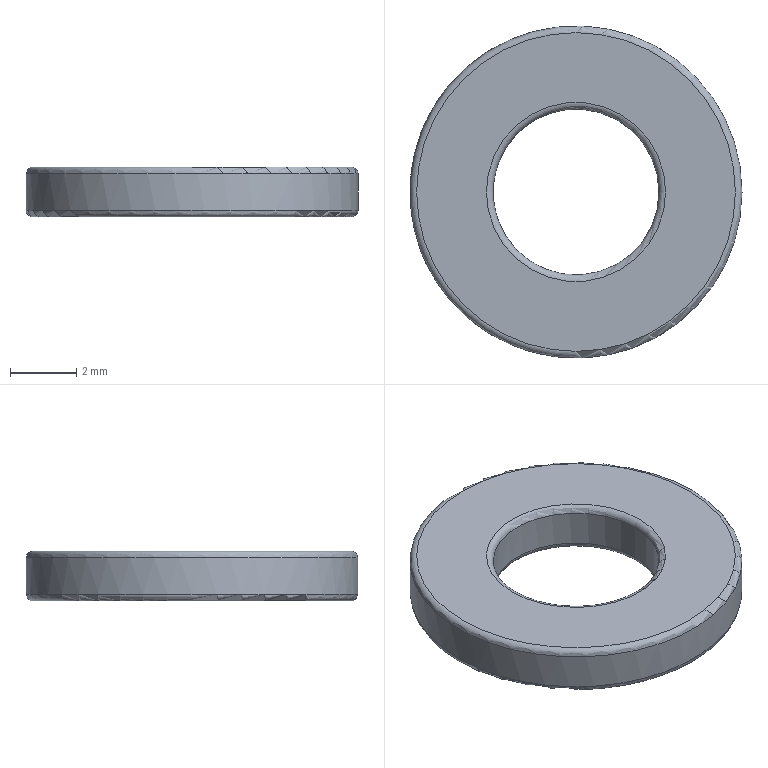Component | NX | MOUNTINGWASHER | 1 solid | 8 faces | box 10 x 10 x 1.5 mm | volume 88 mm3 | torus 4 | plane 2 | cylinder 2 | commonest cylinder face diameters 10 x1 5 x1
STEP:
#1=CARTESIAN_POINT('',(0.,0.,0.));
#2=DIRECTION('',(0.,0.,1.));
#3=DIRECTION('',(1.,0.,0.));
#4=AXIS2_PLACEMENT_3D('',#1,#2,#3);
#5=CARTESIAN_POINT('',(-465.,-20.638,-6.5));
#6=VERTEX_POINT('',#5);
#7=CARTESIAN_POINT('',(-462.3,-20.638,-6.5));
#8=DIRECTION('',(0.,0.,1.));
#9=DIRECTION('',(-1.,0.,0.));
#10=AXIS2_PLACEMENT_3D('',#7,#8,#9);
#11=CIRCLE('',#10,2.7);
#12=CARTESIAN_POINT('',(-462.3,-20.638,-6.5));
#13=DIRECTION('',(0.,0.,-1.));
#14=DIRECTION('',(-1.,0.,0.));
#15=AXIS2_PLACEMENT_3D('',#12,#13,#14);
#16=PLANE('',#15);
#17=CARTESIAN_POINT('',(2.7,0.));
#18=CARTESIAN_POINT('',(2.7,-4.677));
#19=CARTESIAN_POINT('',(-1.35,-2.338));
#20=CARTESIAN_POINT('',(-5.4,-0.));
#21=CARTESIAN_POINT('',(-1.35,2.338));
#22=CARTESIAN_POINT('',(2.7,4.677));
#23=CARTESIAN_POINT('',(2.7,0.));
#24=(BOUNDED_CURVE()B_SPLINE_CURVE(2,(#17,#18,#19,#20,#21,#22,#23),.UNSPECIFIED.,.T.,.F.)B_SPLINE_CURVE_WITH_KNOTS((1,2,2,2,2,1),(-2.094,0.,2.094,4.189,6.283,8.378),.UNSPECIFIED.)CURVE()GEOMETRIC_REPRESENTATION_ITEM()RATIONAL_B_SPLINE_CURVE((1.,0.5,1.,0.5,1.,0.5,1.))REPRESENTATION_ITEM(''));
#25=(GEOMETRIC_REPRESENTATION_CONTEXT(2)PARAMETRIC_REPRESENTATION_CONTEXT()REPRESENTATION_CONTEXT('',''));
#26=DEFINITIONAL_REPRESENTATION('',(#24),#25);
#27=PCURVE('',#16,#26);
#28=CARTESIAN_POINT('',(-462.3,-20.638,-6.3));
#29=DIRECTION('',(0.,0.,-1.));
#30=DIRECTION('',(-1.,0.,0.));
#31=AXIS2_PLACEMENT_3D('',#28,#29,#30);
#32=TOROIDAL_SURFACE('',#31,2.7,0.2);
#33=CARTESIAN_POINT('',(6.283,7.854));
#34=DIRECTION('',(-1.,0.));
#35=VECTOR('',#34,1.);
#36=LINE('',#33,#35);
#37=(GEOMETRIC_REPRESENTATION_CONTEXT(2)PARAMETRIC_REPRESENTATION_CONTEXT()REPRESENTATION_CONTEXT('',''));
#38=DEFINITIONAL_REPRESENTATION('',(#36),#37);
#39=PCURVE('',#32,#38);
#40=SURFACE_CURVE('',#11,(#27,#39),.PCURVE_S1.);
#41=EDGE_CURVE('',#6,#6,#40,.T.);
#42=ORIENTED_EDGE('',*,*,#41,.T.);
#43=EDGE_LOOP('',(#42));
#44=FACE_BOUND('',#43,.T.);
#45=CARTESIAN_POINT('',(-467.1,-20.638,-6.5));
#46=VERTEX_POINT('',#45);
#47=CARTESIAN_POINT('',(-462.3,-20.638,-6.5));
#48=DIRECTION('',(0.,0.,-1.));
#49=DIRECTION('',(-1.,0.,0.));
#50=AXIS2_PLACEMENT_3D('',#47,#48,#49);
#51=CIRCLE('',#50,4.8);
#52=CARTESIAN_POINT('',(0.,0.));
#53=DIRECTION('',(1.,0.));
#54=AXIS2_PLACEMENT_2D('',#52,#53);
#55=CIRCLE('',#54,4.8);
#56=(GEOMETRIC_REPRESENTATION_CONTEXT(2)PARAMETRIC_REPRESENTATION_CONTEXT()REPRESENTATION_CONTEXT('',''));
#57=DEFINITIONAL_REPRESENTATION('',(#55),#56);
#58=PCURVE('',#16,#57);
#59=CARTESIAN_POINT('',(-462.3,-20.638,-6.3));
#60=DIRECTION('',(0.,0.,-1.));
#61=DIRECTION('',(-1.,0.,0.));
#62=AXIS2_PLACEMENT_3D('',#59,#60,#61);
#63=TOROIDAL_SURFACE('',#62,4.8,0.2);
#64=CARTESIAN_POINT('',(0.,7.854));
#65=DIRECTION('',(1.,0.));
#66=VECTOR('',#65,1.);
#67=LINE('',#64,#66);
#68=(GEOMETRIC_REPRESENTATION_CONTEXT(2)PARAMETRIC_REPRESENTATION_CONTEXT()REPRESENTATION_CONTEXT('',''));
#69=DEFINITIONAL_REPRESENTATION('',(#67),#68);
#70=PCURVE('',#63,#69);
#71=SURFACE_CURVE('',#51,(#58,#70),.PCURVE_S1.);
#72=EDGE_CURVE('',#46,#46,#71,.T.);
#73=ORIENTED_EDGE('',*,*,#72,.T.);
#74=EDGE_LOOP('',(#73));
#75=FACE_BOUND('',#74,.T.);
#76=ADVANCED_FACE('',(#44,#75),#16,.T.);
#77=CARTESIAN_POINT('',(-459.6,-20.638,-5.));
#78=VERTEX_POINT('',#77);
#79=CARTESIAN_POINT('',(-462.3,-20.638,-5.));
#80=DIRECTION('',(0.,0.,-1.));
#81=DIRECTION('',(1.,0.,0.));
#82=AXIS2_PLACEMENT_3D('',#79,#80,#81);
#83=CIRCLE('',#82,2.7);
#84=CARTESIAN_POINT('',(-462.3,-20.638,-5.));
#85=DIRECTION('',(0.,0.,1.));
#86=DIRECTION('',(1.,0.,0.));
#87=AXIS2_PLACEMENT_3D('',#84,#85,#86);
#88=PLANE('',#87);
#89=CARTESIAN_POINT('',(2.7,0.));
#90=CARTESIAN_POINT('',(2.7,-4.677));
#91=CARTESIAN_POINT('',(-1.35,-2.338));
#92=CARTESIAN_POINT('',(-5.4,-0.));
#93=CARTESIAN_POINT('',(-1.35,2.338));
#94=CARTESIAN_POINT('',(2.7,4.677));
#95=CARTESIAN_POINT('',(2.7,0.));
#96=(BOUNDED_CURVE()B_SPLINE_CURVE(2,(#89,#90,#91,#92,#93,#94,#95),.UNSPECIFIED.,.T.,.F.)B_SPLINE_CURVE_WITH_KNOTS((1,2,2,2,2,1),(-2.094,0.,2.094,4.189,6.283,8.378),.UNSPECIFIED.)CURVE()GEOMETRIC_REPRESENTATION_ITEM()RATIONAL_B_SPLINE_CURVE((1.,0.5,1.,0.5,1.,0.5,1.))REPRESENTATION_ITEM(''));
#97=(GEOMETRIC_REPRESENTATION_CONTEXT(2)PARAMETRIC_REPRESENTATION_CONTEXT()REPRESENTATION_CONTEXT('',''));
#98=DEFINITIONAL_REPRESENTATION('',(#96),#97);
#99=PCURVE('',#88,#98);
#100=CARTESIAN_POINT('',(-462.3,-20.638,-5.2));
#101=DIRECTION('',(0.,0.,1.));
#102=DIRECTION('',(1.,0.,0.));
#103=AXIS2_PLACEMENT_3D('',#100,#101,#102);
#104=TOROIDAL_SURFACE('',#103,2.7,0.2);
#105=CARTESIAN_POINT('',(6.283,7.854));
#106=DIRECTION('',(-1.,0.));
#107=VECTOR('',#106,1.);
#108=LINE('',#105,#107);
#109=(GEOMETRIC_REPRESENTATION_CONTEXT(2)PARAMETRIC_REPRESENTATION_CONTEXT()REPRESENTATION_CONTEXT('',''));
#110=DEFINITIONAL_REPRESENTATION('',(#108),#109);
#111=PCURVE('',#104,#110);
#112=SURFACE_CURVE('',#83,(#99,#111),.PCURVE_S1.);
#113=EDGE_CURVE('',#78,#78,#112,.T.);
#114=ORIENTED_EDGE('',*,*,#113,.T.);
#115=EDGE_LOOP('',(#114));
#116=FACE_BOUND('',#115,.T.);
#117=CARTESIAN_POINT('',(-457.5,-20.638,-5.));
#118=VERTEX_POINT('',#117);
#119=CARTESIAN_POINT('',(-462.3,-20.638,-5.));
#120=DIRECTION('',(0.,0.,1.));
#121=DIRECTION('',(1.,0.,0.));
#122=AXIS2_PLACEMENT_3D('',#119,#120,#121);
#123=CIRCLE('',#122,4.8);
#124=CARTESIAN_POINT('',(0.,0.));
#125=DIRECTION('',(1.,0.));
#126=AXIS2_PLACEMENT_2D('',#124,#125);
#127=CIRCLE('',#126,4.8);
#128=(GEOMETRIC_REPRESENTATION_CONTEXT(2)PARAMETRIC_REPRESENTATION_CONTEXT()REPRESENTATION_CONTEXT('',''));
#129=DEFINITIONAL_REPRESENTATION('',(#127),#128);
#130=PCURVE('',#88,#129);
#131=CARTESIAN_POINT('',(-462.3,-20.638,-5.2));
#132=DIRECTION('',(0.,0.,1.));
#133=DIRECTION('',(1.,0.,0.));
#134=AXIS2_PLACEMENT_3D('',#131,#132,#133);
#135=TOROIDAL_SURFACE('',#134,4.8,0.2);
#136=CARTESIAN_POINT('',(0.,7.854));
#137=DIRECTION('',(1.,0.));
#138=VECTOR('',#137,1.);
#139=LINE('',#136,#138);
#140=(GEOMETRIC_REPRESENTATION_CONTEXT(2)PARAMETRIC_REPRESENTATION_CONTEXT()REPRESENTATION_CONTEXT('',''));
#141=DEFINITIONAL_REPRESENTATION('',(#139),#140);
#142=PCURVE('',#135,#141);
#143=SURFACE_CURVE('',#123,(#130,#142),.PCURVE_S1.);
#144=EDGE_CURVE('',#118,#118,#143,.T.);
#145=ORIENTED_EDGE('',*,*,#144,.T.);
#146=EDGE_LOOP('',(#145));
#147=FACE_BOUND('',#146,.T.);
#148=ADVANCED_FACE('',(#116,#147),#88,.T.);
#149=CARTESIAN_POINT('',(-457.3,-20.638,-5.2));
#150=VERTEX_POINT('',#149);
#151=CARTESIAN_POINT('',(-462.3,-20.638,-5.2));
#152=DIRECTION('',(0.,0.,-1.));
#153=DIRECTION('',(1.,0.,0.));
#154=AXIS2_PLACEMENT_3D('',#151,#152,#153);
#155=CIRCLE('',#154,5.);
#156=CARTESIAN_POINT('',(-462.3,-20.638,-5.));
#157=DIRECTION('',(0.,0.,-1.));
#158=DIRECTION('',(1.,0.,0.));
#159=AXIS2_PLACEMENT_3D('',#156,#157,#158);
#160=CYLINDRICAL_SURFACE('',#159,5.);
#161=CARTESIAN_POINT('',(0.,0.2));
#162=DIRECTION('',(1.,0.));
#163=VECTOR('',#162,1.);
#164=LINE('',#161,#163);
#165=(GEOMETRIC_REPRESENTATION_CONTEXT(2)PARAMETRIC_REPRESENTATION_CONTEXT()REPRESENTATION_CONTEXT('',''));
#166=DEFINITIONAL_REPRESENTATION('',(#164),#165);
#167=PCURVE('',#160,#166);
#168=CARTESIAN_POINT('',(6.283,6.283));
#169=DIRECTION('',(-1.,0.));
#170=VECTOR('',#169,1.);
#171=LINE('',#168,#170);
#172=(GEOMETRIC_REPRESENTATION_CONTEXT(2)PARAMETRIC_REPRESENTATION_CONTEXT()REPRESENTATION_CONTEXT('',''));
#173=DEFINITIONAL_REPRESENTATION('',(#171),#172);
#174=PCURVE('',#135,#173);
#175=SURFACE_CURVE('',#155,(#167,#174),.PCURVE_S1.);
#176=EDGE_CURVE('',#150,#150,#175,.T.);
#177=ORIENTED_EDGE('',*,*,#176,.T.);
#178=CARTESIAN_POINT('',(-457.3,-20.638,-6.3));
#179=VERTEX_POINT('',#178);
#180=CARTESIAN_POINT('',(-457.3,-20.638,-5.2));
#181=CARTESIAN_POINT('',(-457.3,-20.638,-6.3));
#182=B_SPLINE_CURVE_WITH_KNOTS('',1,(#180,#181),.UNSPECIFIED.,.F.,.F.,(2,2),(0.2,1.3),.PIECEWISE_BEZIER_KNOTS.);
#183=CARTESIAN_POINT('',(6.283,0.));
#184=DIRECTION('',(0.,1.));
#185=VECTOR('',#184,1.);
#186=LINE('',#183,#185);
#187=(GEOMETRIC_REPRESENTATION_CONTEXT(2)PARAMETRIC_REPRESENTATION_CONTEXT()REPRESENTATION_CONTEXT('',''));
#188=DEFINITIONAL_REPRESENTATION('',(#186),#187);
#189=PCURVE('',#160,#188);
#190=CARTESIAN_POINT('',(0.,0.));
#191=DIRECTION('',(0.,1.));
#192=VECTOR('',#191,1.);
#193=LINE('',#190,#192);
#194=(GEOMETRIC_REPRESENTATION_CONTEXT(2)PARAMETRIC_REPRESENTATION_CONTEXT()REPRESENTATION_CONTEXT('',''));
#195=DEFINITIONAL_REPRESENTATION('',(#193),#194);
#196=PCURVE('',#160,#195);
#197=SEAM_CURVE('',#182,(#189,#196),.PCURVE_S1.);
#198=EDGE_CURVE('',#150,#179,#197,.T.);
#199=ORIENTED_EDGE('',*,*,#198,.T.);
#200=CARTESIAN_POINT('',(-467.3,-20.638,-6.3));
#201=VERTEX_POINT('',#200);
#202=CARTESIAN_POINT('',(-462.3,-20.638,-6.3));
#203=DIRECTION('',(0.,0.,1.));
#204=DIRECTION('',(-1.,0.,0.));
#205=AXIS2_PLACEMENT_3D('',#202,#203,#204);
#206=CIRCLE('',#205,5.);
#207=CARTESIAN_POINT('',(9.425,1.3));
#208=DIRECTION('',(-1.,0.));
#209=VECTOR('',#208,1.);
#210=LINE('',#207,#209);
#211=(GEOMETRIC_REPRESENTATION_CONTEXT(2)PARAMETRIC_REPRESENTATION_CONTEXT()REPRESENTATION_CONTEXT('',''));
#212=DEFINITIONAL_REPRESENTATION('',(#210),#211);
#213=PCURVE('',#160,#212);
#214=CARTESIAN_POINT('',(6.283,6.283));
#215=DIRECTION('',(-1.,0.));
#216=VECTOR('',#215,1.);
#217=LINE('',#214,#216);
#218=(GEOMETRIC_REPRESENTATION_CONTEXT(2)PARAMETRIC_REPRESENTATION_CONTEXT()REPRESENTATION_CONTEXT('',''));
#219=DEFINITIONAL_REPRESENTATION('',(#217),#218);
#220=PCURVE('',#63,#219);
#221=SURFACE_CURVE('',#206,(#213,#220),.PCURVE_S1.);
#222=EDGE_CURVE('',#179,#201,#221,.T.);
#223=ORIENTED_EDGE('',*,*,#222,.T.);
#224=CARTESIAN_POINT('',(-462.3,-20.638,-6.3));
#225=DIRECTION('',(0.,0.,1.));
#226=DIRECTION('',(-1.,0.,0.));
#227=AXIS2_PLACEMENT_3D('',#224,#225,#226);
#228=CIRCLE('',#227,5.);
#229=CARTESIAN_POINT('',(3.142,1.3));
#230=DIRECTION('',(-1.,0.));
#231=VECTOR('',#230,1.);
#232=LINE('',#229,#231);
#233=(GEOMETRIC_REPRESENTATION_CONTEXT(2)PARAMETRIC_REPRESENTATION_CONTEXT()REPRESENTATION_CONTEXT('',''));
#234=DEFINITIONAL_REPRESENTATION('',(#232),#233);
#235=PCURVE('',#160,#234);
#236=CARTESIAN_POINT('',(6.283,6.283));
#237=DIRECTION('',(-1.,0.));
#238=VECTOR('',#237,1.);
#239=LINE('',#236,#238);
#240=(GEOMETRIC_REPRESENTATION_CONTEXT(2)PARAMETRIC_REPRESENTATION_CONTEXT()REPRESENTATION_CONTEXT('',''));
#241=DEFINITIONAL_REPRESENTATION('',(#239),#240);
#242=PCURVE('',#63,#241);
#243=SURFACE_CURVE('',#228,(#235,#242),.PCURVE_S1.);
#244=EDGE_CURVE('',#201,#179,#243,.T.);
#245=ORIENTED_EDGE('',*,*,#244,.T.);
#246=ORIENTED_EDGE('',*,*,#198,.F.);
#247=EDGE_LOOP('',(#177,#199,#223,#245,#246));
#248=FACE_BOUND('',#247,.T.);
#249=ADVANCED_FACE('',(#248),#160,.T.);
#250=CARTESIAN_POINT('',(-459.8,-20.638,-6.3));
#251=VERTEX_POINT('',#250);
#252=CARTESIAN_POINT('',(-464.8,-20.638,-6.3));
#253=VERTEX_POINT('',#252);
#254=CARTESIAN_POINT('',(-462.3,-20.638,-6.3));
#255=DIRECTION('',(0.,0.,-1.));
#256=DIRECTION('',(-1.,0.,0.));
#257=AXIS2_PLACEMENT_3D('',#254,#255,#256);
#258=CIRCLE('',#257,2.5);
#259=CARTESIAN_POINT('',(-462.3,-20.638,-6.5));
#260=DIRECTION('',(0.,0.,1.));
#261=DIRECTION('',(1.,0.,0.));
#262=AXIS2_PLACEMENT_3D('',#259,#260,#261);
#263=CYLINDRICAL_SURFACE('',#262,2.5);
#264=CARTESIAN_POINT('',(9.425,0.2));
#265=DIRECTION('',(-1.,0.));
#266=VECTOR('',#265,1.);
#267=LINE('',#264,#266);
#268=(GEOMETRIC_REPRESENTATION_CONTEXT(2)PARAMETRIC_REPRESENTATION_CONTEXT()REPRESENTATION_CONTEXT('',''));
#269=DEFINITIONAL_REPRESENTATION('',(#267),#268);
#270=PCURVE('',#263,#269);
#271=CARTESIAN_POINT('',(0.,9.425));
#272=DIRECTION('',(1.,0.));
#273=VECTOR('',#272,1.);
#274=LINE('',#271,#273);
#275=(GEOMETRIC_REPRESENTATION_CONTEXT(2)PARAMETRIC_REPRESENTATION_CONTEXT()REPRESENTATION_CONTEXT('',''));
#276=DEFINITIONAL_REPRESENTATION('',(#274),#275);
#277=PCURVE('',#32,#276);
#278=SURFACE_CURVE('',#258,(#270,#277),.PCURVE_S1.);
#279=EDGE_CURVE('',#251,#253,#278,.T.);
#280=ORIENTED_EDGE('',*,*,#279,.F.);
#281=CARTESIAN_POINT('',(-459.8,-20.638,-5.2));
#282=VERTEX_POINT('',#281);
#283=CARTESIAN_POINT('',(-459.8,-20.638,-6.3));
#284=CARTESIAN_POINT('',(-459.8,-20.638,-5.2));
#285=B_SPLINE_CURVE_WITH_KNOTS('',1,(#283,#284),.UNSPECIFIED.,.F.,.F.,(2,2),(0.2,1.3),.PIECEWISE_BEZIER_KNOTS.);
#286=CARTESIAN_POINT('',(6.283,0.));
#287=DIRECTION('',(0.,1.));
#288=VECTOR('',#287,1.);
#289=LINE('',#286,#288);
#290=(GEOMETRIC_REPRESENTATION_CONTEXT(2)PARAMETRIC_REPRESENTATION_CONTEXT()REPRESENTATION_CONTEXT('',''));
#291=DEFINITIONAL_REPRESENTATION('',(#289),#290);
#292=PCURVE('',#263,#291);
#293=CARTESIAN_POINT('',(0.,0.));
#294=DIRECTION('',(0.,1.));
#295=VECTOR('',#294,1.);
#296=LINE('',#293,#295);
#297=(GEOMETRIC_REPRESENTATION_CONTEXT(2)PARAMETRIC_REPRESENTATION_CONTEXT()REPRESENTATION_CONTEXT('',''));
#298=DEFINITIONAL_REPRESENTATION('',(#296),#297);
#299=PCURVE('',#263,#298);
#300=SEAM_CURVE('',#285,(#292,#299),.PCURVE_S1.);
#301=EDGE_CURVE('',#251,#282,#300,.T.);
#302=ORIENTED_EDGE('',*,*,#301,.T.);
#303=CARTESIAN_POINT('',(-462.3,-20.638,-5.2));
#304=DIRECTION('',(0.,0.,1.));
#305=DIRECTION('',(1.,0.,0.));
#306=AXIS2_PLACEMENT_3D('',#303,#304,#305);
#307=CIRCLE('',#306,2.5);
#308=CARTESIAN_POINT('',(0.,1.3));
#309=DIRECTION('',(1.,0.));
#310=VECTOR('',#309,1.);
#311=LINE('',#308,#310);
#312=(GEOMETRIC_REPRESENTATION_CONTEXT(2)PARAMETRIC_REPRESENTATION_CONTEXT()REPRESENTATION_CONTEXT('',''));
#313=DEFINITIONAL_REPRESENTATION('',(#311),#312);
#314=PCURVE('',#263,#313);
#315=CARTESIAN_POINT('',(0.,9.425));
#316=DIRECTION('',(1.,0.));
#317=VECTOR('',#316,1.);
#318=LINE('',#315,#317);
#319=(GEOMETRIC_REPRESENTATION_CONTEXT(2)PARAMETRIC_REPRESENTATION_CONTEXT()REPRESENTATION_CONTEXT('',''));
#320=DEFINITIONAL_REPRESENTATION('',(#318),#319);
#321=PCURVE('',#104,#320);
#322=SURFACE_CURVE('',#307,(#314,#321),.PCURVE_S1.);
#323=EDGE_CURVE('',#282,#282,#322,.T.);
#324=ORIENTED_EDGE('',*,*,#323,.F.);
#325=ORIENTED_EDGE('',*,*,#301,.F.);
#326=CARTESIAN_POINT('',(-462.3,-20.638,-6.3));
#327=DIRECTION('',(0.,0.,-1.));
#328=DIRECTION('',(-1.,0.,0.));
#329=AXIS2_PLACEMENT_3D('',#326,#327,#328);
#330=CIRCLE('',#329,2.5);
#331=CARTESIAN_POINT('',(3.142,0.2));
#332=DIRECTION('',(-1.,0.));
#333=VECTOR('',#332,1.);
#334=LINE('',#331,#333);
#335=(GEOMETRIC_REPRESENTATION_CONTEXT(2)PARAMETRIC_REPRESENTATION_CONTEXT()REPRESENTATION_CONTEXT('',''));
#336=DEFINITIONAL_REPRESENTATION('',(#334),#335);
#337=PCURVE('',#263,#336);
#338=CARTESIAN_POINT('',(0.,9.425));
#339=DIRECTION('',(1.,-0.));
#340=VECTOR('',#339,1.);
#341=LINE('',#338,#340);
#342=(GEOMETRIC_REPRESENTATION_CONTEXT(2)PARAMETRIC_REPRESENTATION_CONTEXT()REPRESENTATION_CONTEXT('',''));
#343=DEFINITIONAL_REPRESENTATION('',(#341),#342);
#344=PCURVE('',#32,#343);
#345=SURFACE_CURVE('',#330,(#337,#344),.PCURVE_S1.);
#346=EDGE_CURVE('',#253,#251,#345,.T.);
#347=ORIENTED_EDGE('',*,*,#346,.F.);
#348=EDGE_LOOP('',(#280,#302,#324,#325,#347));
#349=FACE_BOUND('',#348,.F.);
#350=ADVANCED_FACE('',(#349),#263,.F.);
#351=ORIENTED_EDGE('',*,*,#346,.F.);
#352=CARTESIAN_POINT('',(-465.,-20.638,-6.5));
#353=CARTESIAN_POINT('',(-464.947,-20.638,-6.5));
#354=CARTESIAN_POINT('',(-464.894,-20.638,-6.483));
#355=CARTESIAN_POINT('',(-464.85,-20.638,-6.45));
#356=CARTESIAN_POINT('',(-464.817,-20.638,-6.406));
#357=CARTESIAN_POINT('',(-464.8,-20.638,-6.353));
#358=CARTESIAN_POINT('',(-464.8,-20.638,-6.3));
#359=(BOUNDED_CURVE()B_SPLINE_CURVE(6,(#352,#353,#354,#355,#356,#357,#358),.UNSPECIFIED.,.F.,.F.)B_SPLINE_CURVE_WITH_KNOTS((7,7),(1.571,3.142),.PIECEWISE_BEZIER_KNOTS.)CURVE()GEOMETRIC_REPRESENTATION_ITEM()RATIONAL_B_SPLINE_CURVE((1.031,1.01,0.9979,0.994,0.9979,1.01,1.031))REPRESENTATION_ITEM(''));
#360=CARTESIAN_POINT('',(0.,6.283));
#361=DIRECTION('',(0.,1.));
#362=VECTOR('',#361,1.);
#363=LINE('',#360,#362);
#364=(GEOMETRIC_REPRESENTATION_CONTEXT(2)PARAMETRIC_REPRESENTATION_CONTEXT()REPRESENTATION_CONTEXT('',''));
#365=DEFINITIONAL_REPRESENTATION('',(#363),#364);
#366=PCURVE('',#32,#365);
#367=CARTESIAN_POINT('',(6.283,6.283));
#368=DIRECTION('',(0.,1.));
#369=VECTOR('',#368,1.);
#370=LINE('',#367,#369);
#371=(GEOMETRIC_REPRESENTATION_CONTEXT(2)PARAMETRIC_REPRESENTATION_CONTEXT()REPRESENTATION_CONTEXT('',''));
#372=DEFINITIONAL_REPRESENTATION('',(#370),#371);
#373=PCURVE('',#32,#372);
#374=SEAM_CURVE('',#359,(#366,#373),.PCURVE_S1.);
#375=EDGE_CURVE('',#6,#253,#374,.T.);
#376=ORIENTED_EDGE('',*,*,#375,.F.);
#377=ORIENTED_EDGE('',*,*,#41,.F.);
#378=ORIENTED_EDGE('',*,*,#375,.T.);
#379=ORIENTED_EDGE('',*,*,#279,.F.);
#380=EDGE_LOOP('',(#351,#376,#377,#378,#379));
#381=FACE_BOUND('',#380,.T.);
#382=ADVANCED_FACE('',(#381),#32,.T.);
#383=ORIENTED_EDGE('',*,*,#323,.F.);
#384=CARTESIAN_POINT('',(-459.6,-20.638,-5.));
#385=CARTESIAN_POINT('',(-459.653,-20.638,-5.));
#386=CARTESIAN_POINT('',(-459.706,-20.638,-5.017));
#387=CARTESIAN_POINT('',(-459.75,-20.638,-5.05));
#388=CARTESIAN_POINT('',(-459.783,-20.638,-5.094));
#389=CARTESIAN_POINT('',(-459.8,-20.638,-5.147));
#390=CARTESIAN_POINT('',(-459.8,-20.638,-5.2));
#391=(BOUNDED_CURVE()B_SPLINE_CURVE(6,(#384,#385,#386,#387,#388,#389,#390),.UNSPECIFIED.,.F.,.F.)B_SPLINE_CURVE_WITH_KNOTS((7,7),(1.571,3.142),.PIECEWISE_BEZIER_KNOTS.)CURVE()GEOMETRIC_REPRESENTATION_ITEM()RATIONAL_B_SPLINE_CURVE((1.031,1.01,0.9979,0.994,0.9979,1.01,1.031))REPRESENTATION_ITEM(''));
#392=CARTESIAN_POINT('',(0.,6.283));
#393=DIRECTION('',(0.,1.));
#394=VECTOR('',#393,1.);
#395=LINE('',#392,#394);
#396=(GEOMETRIC_REPRESENTATION_CONTEXT(2)PARAMETRIC_REPRESENTATION_CONTEXT()REPRESENTATION_CONTEXT('',''));
#397=DEFINITIONAL_REPRESENTATION('',(#395),#396);
#398=PCURVE('',#104,#397);
#399=CARTESIAN_POINT('',(6.283,6.283));
#400=DIRECTION('',(0.,1.));
#401=VECTOR('',#400,1.);
#402=LINE('',#399,#401);
#403=(GEOMETRIC_REPRESENTATION_CONTEXT(2)PARAMETRIC_REPRESENTATION_CONTEXT()REPRESENTATION_CONTEXT('',''));
#404=DEFINITIONAL_REPRESENTATION('',(#402),#403);
#405=PCURVE('',#104,#404);
#406=SEAM_CURVE('',#391,(#398,#405),.PCURVE_S1.);
#407=EDGE_CURVE('',#78,#282,#406,.T.);
#408=ORIENTED_EDGE('',*,*,#407,.F.);
#409=ORIENTED_EDGE('',*,*,#113,.F.);
#410=ORIENTED_EDGE('',*,*,#407,.T.);
#411=EDGE_LOOP('',(#383,#408,#409,#410));
#412=FACE_BOUND('',#411,.T.);
#413=ADVANCED_FACE('',(#412),#104,.T.);
#414=ORIENTED_EDGE('',*,*,#144,.F.);
#415=CARTESIAN_POINT('',(-457.3,-20.638,-5.2));
#416=CARTESIAN_POINT('',(-457.3,-20.638,-5.147));
#417=CARTESIAN_POINT('',(-457.317,-20.638,-5.094));
#418=CARTESIAN_POINT('',(-457.35,-20.638,-5.05));
#419=CARTESIAN_POINT('',(-457.394,-20.638,-5.017));
#420=CARTESIAN_POINT('',(-457.447,-20.638,-5.));
#421=CARTESIAN_POINT('',(-457.5,-20.638,-5.));
#422=(BOUNDED_CURVE()B_SPLINE_CURVE(6,(#415,#416,#417,#418,#419,#420,#421),.UNSPECIFIED.,.F.,.F.)B_SPLINE_CURVE_WITH_KNOTS((7,7),(0.,1.571),.PIECEWISE_BEZIER_KNOTS.)CURVE()GEOMETRIC_REPRESENTATION_ITEM()RATIONAL_B_SPLINE_CURVE((1.031,1.01,0.9979,0.994,0.9979,1.01,1.031))REPRESENTATION_ITEM(''));
#423=CARTESIAN_POINT('',(0.,6.283));
#424=DIRECTION('',(0.,1.));
#425=VECTOR('',#424,1.);
#426=LINE('',#423,#425);
#427=(GEOMETRIC_REPRESENTATION_CONTEXT(2)PARAMETRIC_REPRESENTATION_CONTEXT()REPRESENTATION_CONTEXT('',''));
#428=DEFINITIONAL_REPRESENTATION('',(#426),#427);
#429=PCURVE('',#135,#428);
#430=CARTESIAN_POINT('',(6.283,6.283));
#431=DIRECTION('',(0.,1.));
#432=VECTOR('',#431,1.);
#433=LINE('',#430,#432);
#434=(GEOMETRIC_REPRESENTATION_CONTEXT(2)PARAMETRIC_REPRESENTATION_CONTEXT()REPRESENTATION_CONTEXT('',''));
#435=DEFINITIONAL_REPRESENTATION('',(#433),#434);
#436=PCURVE('',#135,#435);
#437=SEAM_CURVE('',#422,(#429,#436),.PCURVE_S1.);
#438=EDGE_CURVE('',#150,#118,#437,.T.);
#439=ORIENTED_EDGE('',*,*,#438,.F.);
#440=ORIENTED_EDGE('',*,*,#176,.F.);
#441=ORIENTED_EDGE('',*,*,#438,.T.);
#442=EDGE_LOOP('',(#414,#439,#440,#441));
#443=FACE_BOUND('',#442,.T.);
#444=ADVANCED_FACE('',(#443),#135,.T.);
#445=ORIENTED_EDGE('',*,*,#72,.F.);
#446=CARTESIAN_POINT('',(-467.3,-20.638,-6.3));
#447=CARTESIAN_POINT('',(-467.3,-20.638,-6.353));
#448=CARTESIAN_POINT('',(-467.283,-20.638,-6.406));
#449=CARTESIAN_POINT('',(-467.25,-20.638,-6.45));
#450=CARTESIAN_POINT('',(-467.206,-20.638,-6.483));
#451=CARTESIAN_POINT('',(-467.153,-20.638,-6.5));
#452=CARTESIAN_POINT('',(-467.1,-20.638,-6.5));
#453=(BOUNDED_CURVE()B_SPLINE_CURVE(6,(#446,#447,#448,#449,#450,#451,#452),.UNSPECIFIED.,.F.,.F.)B_SPLINE_CURVE_WITH_KNOTS((7,7),(0.,1.571),.PIECEWISE_BEZIER_KNOTS.)CURVE()GEOMETRIC_REPRESENTATION_ITEM()RATIONAL_B_SPLINE_CURVE((1.031,1.01,0.9979,0.994,0.9979,1.01,1.031))REPRESENTATION_ITEM(''));
#454=CARTESIAN_POINT('',(0.,6.283));
#455=DIRECTION('',(0.,1.));
#456=VECTOR('',#455,1.);
#457=LINE('',#454,#456);
#458=(GEOMETRIC_REPRESENTATION_CONTEXT(2)PARAMETRIC_REPRESENTATION_CONTEXT()REPRESENTATION_CONTEXT('',''));
#459=DEFINITIONAL_REPRESENTATION('',(#457),#458);
#460=PCURVE('',#63,#459);
#461=CARTESIAN_POINT('',(6.283,6.283));
#462=DIRECTION('',(0.,1.));
#463=VECTOR('',#462,1.);
#464=LINE('',#461,#463);
#465=(GEOMETRIC_REPRESENTATION_CONTEXT(2)PARAMETRIC_REPRESENTATION_CONTEXT()REPRESENTATION_CONTEXT('',''));
#466=DEFINITIONAL_REPRESENTATION('',(#464),#465);
#467=PCURVE('',#63,#466);
#468=SEAM_CURVE('',#453,(#460,#467),.PCURVE_S1.);
#469=EDGE_CURVE('',#201,#46,#468,.T.);
#470=ORIENTED_EDGE('',*,*,#469,.F.);
#471=ORIENTED_EDGE('',*,*,#222,.F.);
#472=ORIENTED_EDGE('',*,*,#244,.F.);
#473=ORIENTED_EDGE('',*,*,#469,.T.);
#474=EDGE_LOOP('',(#445,#470,#471,#472,#473));
#475=FACE_BOUND('',#474,.T.);
#476=ADVANCED_FACE('',(#475),#63,.T.);
#477=CLOSED_SHELL('',(#76,#148,#249,#350,#382,#413,#444,#476));
#478=MANIFOLD_SOLID_BREP('',#477);
#479=(LENGTH_UNIT()NAMED_UNIT(*)SI_UNIT(.MILLI.,.METRE.));
#480=UNCERTAINTY_MEASURE_WITH_UNIT(LENGTH_MEASURE(0.00001),#479,'','');
#481=(NAMED_UNIT(*)PLANE_ANGLE_UNIT()SI_UNIT($,.RADIAN.));
#482=(NAMED_UNIT(*)SI_UNIT($,.STERADIAN.)SOLID_ANGLE_UNIT());
#483=(GEOMETRIC_REPRESENTATION_CONTEXT(3)GLOBAL_UNCERTAINTY_ASSIGNED_CONTEXT((#480))GLOBAL_UNIT_ASSIGNED_CONTEXT((#479,#481,#482))REPRESENTATION_CONTEXT('',''));
#484=ADVANCED_BREP_SHAPE_REPRESENTATION('',(#4,#478),#483);